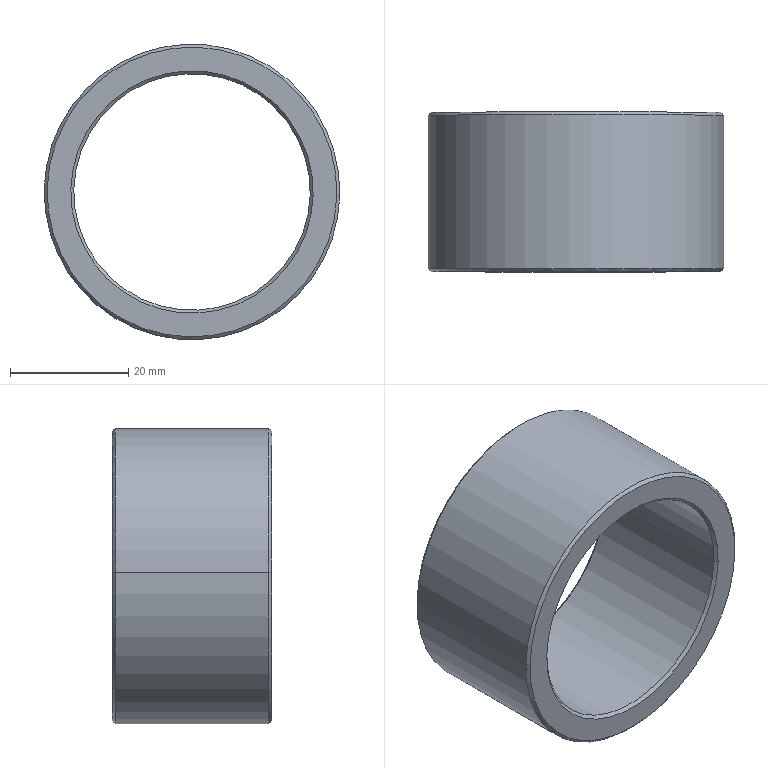Component | SolidWorks | BearingHousingAssembly-1_FixedSleeve-1 | 1 solid | 14 faces | box 50 x 27 x 50 mm | volume 19014 mm3 | cone 8 | cylinder 4 | plane 2 | commonest cylinder face diameters 40 x2 50 x2 | material Plain Carbon Steel
build123d program:
from build123d import *

# Parameters (mm, degrees)
SKETCH1_R           = 25
SKETCH1_R_2         = 20
BOSS_EXTRUDE1_DEPTH = 27
CHAMFER1_SIZE       = 0.5


with BuildPart() as part:
    # Sketch1 → Boss-Extrude1 (new body)
    with BuildSketch(Plane.XY):
        Circle(SKETCH1_R)
        Circle(SKETCH1_R_2, mode=Mode.SUBTRACT)
    extrude(amount=BOSS_EXTRUDE1_DEPTH)

    # Chamfer1
    chamfer1_edges = [part.edges().sort_by_distance(p)[0] for p in [
        (-25, 0, 0),
        (-25, 0, 27),
        (-20, 0, 0),
        (-20, 0, 27),
    ]]
    chamfer(chamfer1_edges, length=CHAMFER1_SIZE)


solid = part.part

# Placed as in the assembly
solid = solid.moved(Location((-38.666, 222.264, -6), (90, 0, 0)))
STEP:
#1=CARTESIAN_POINT('',(-0.558,7.688,-0.2605));
#2=VERTEX_POINT('',#1);
#3=CARTESIAN_POINT('',(-2.487,7.688,-0.2119));
#4=VERTEX_POINT('',#3);
#5=CARTESIAN_POINT('',(-1.522,7.688,-0.2362));
#6=DIRECTION('',(-0.,-1.,-0.));
#7=DIRECTION('',(0.9997,0.,-0.02521));
#8=AXIS2_PLACEMENT_3D('',#5,#6,#7);
#9=CIRCLE('',#8,0.9646);
#10=EDGE_CURVE('',#2,#4,#9,.T.);
#11=ORIENTED_EDGE('',*,*,#10,.F.);
#12=CARTESIAN_POINT('',(-0.5383,7.707,-0.261));
#13=VERTEX_POINT('',#12);
#14=CARTESIAN_POINT('',(-0.558,7.688,-0.2605));
#15=DIRECTION('',(0.7069,0.7071,-0.01783));
#16=VECTOR('',#15,39.37);
#17=LINE('',#14,#16);
#18=EDGE_CURVE('',#2,#13,#17,.T.);
#19=ORIENTED_EDGE('',*,*,#18,.T.);
#20=CARTESIAN_POINT('',(-2.506,7.707,-0.2114));
#21=VERTEX_POINT('',#20);
#22=CARTESIAN_POINT('',(-1.522,7.707,-0.2362));
#23=DIRECTION('',(0.,1.,0.));
#24=DIRECTION('',(0.9997,0.,-0.02521));
#25=AXIS2_PLACEMENT_3D('',#22,#23,#24);
#26=CIRCLE('',#25,0.9843);
#27=EDGE_CURVE('',#21,#13,#26,.T.);
#28=ORIENTED_EDGE('',*,*,#27,.F.);
#29=CARTESIAN_POINT('',(-2.487,7.688,-0.2119));
#30=DIRECTION('',(-0.7069,0.7071,0.01783));
#31=VECTOR('',#30,39.37);
#32=LINE('',#29,#31);
#33=EDGE_CURVE('',#4,#21,#32,.T.);
#34=ORIENTED_EDGE('',*,*,#33,.F.);
#35=EDGE_LOOP('',(#11,#19,#28,#34));
#36=FACE_OUTER_BOUND('',#35,.T.);
#37=CARTESIAN_POINT('',(-1.522,7.688,-0.2362));
#38=DIRECTION('',(0.,1.,0.));
#39=DIRECTION('',(-0.9997,0.,0.02521));
#40=AXIS2_PLACEMENT_3D('',#37,#38,#39);
#41=CONICAL_SURFACE('',#40,0.9646,0.7854);
#42=ADVANCED_FACE('',(#36),#41,.T.);
#43=CARTESIAN_POINT('',(-2.309,7.707,-0.2164));
#44=VERTEX_POINT('',#43);
#45=CARTESIAN_POINT('',(-0.7351,7.707,-0.2561));
#46=VERTEX_POINT('',#45);
#47=CARTESIAN_POINT('',(-1.522,7.707,-0.2362));
#48=DIRECTION('',(-0.,-1.,-0.));
#49=DIRECTION('',(0.9997,0.,-0.02521));
#50=AXIS2_PLACEMENT_3D('',#47,#48,#49);
#51=CIRCLE('',#50,0.7874);
#52=EDGE_CURVE('',#44,#46,#51,.T.);
#53=ORIENTED_EDGE('',*,*,#52,.F.);
#54=CARTESIAN_POINT('',(-2.329,7.688,-0.2159));
#55=VERTEX_POINT('',#54);
#56=CARTESIAN_POINT('',(-2.309,7.707,-0.2164));
#57=DIRECTION('',(-0.7069,-0.7071,0.01783));
#58=VECTOR('',#57,39.37);
#59=LINE('',#56,#58);
#60=EDGE_CURVE('',#44,#55,#59,.T.);
#61=ORIENTED_EDGE('',*,*,#60,.T.);
#62=CARTESIAN_POINT('',(-0.7154,7.688,-0.2566));
#63=VERTEX_POINT('',#62);
#64=CARTESIAN_POINT('',(-1.522,7.688,-0.2362));
#65=DIRECTION('',(0.,1.,0.));
#66=DIRECTION('',(0.9997,0.,-0.02521));
#67=AXIS2_PLACEMENT_3D('',#64,#65,#66);
#68=CIRCLE('',#67,0.8071);
#69=EDGE_CURVE('',#63,#55,#68,.T.);
#70=ORIENTED_EDGE('',*,*,#69,.F.);
#71=CARTESIAN_POINT('',(-0.7351,7.707,-0.2561));
#72=DIRECTION('',(0.7069,-0.7071,-0.01783));
#73=VECTOR('',#72,39.37);
#74=LINE('',#71,#73);
#75=EDGE_CURVE('',#46,#63,#74,.T.);
#76=ORIENTED_EDGE('',*,*,#75,.F.);
#77=EDGE_LOOP('',(#53,#61,#70,#76));
#78=FACE_OUTER_BOUND('',#77,.T.);
#79=CARTESIAN_POINT('',(-1.522,7.707,-0.2362));
#80=DIRECTION('',(-0.,-1.,-0.));
#81=DIRECTION('',(0.9997,0.,-0.02521));
#82=AXIS2_PLACEMENT_3D('',#79,#80,#81);
#83=CONICAL_SURFACE('',#82,0.7874,0.7854);
#84=ADVANCED_FACE('',(#78),#83,.F.);
#85=CARTESIAN_POINT('',(-0.7351,8.731,-0.2561));
#86=VERTEX_POINT('',#85);
#87=CARTESIAN_POINT('',(-2.309,8.731,-0.2164));
#88=VERTEX_POINT('',#87);
#89=CARTESIAN_POINT('',(-1.522,8.731,-0.2362));
#90=DIRECTION('',(0.,1.,0.));
#91=DIRECTION('',(0.9997,0.,-0.02521));
#92=AXIS2_PLACEMENT_3D('',#89,#90,#91);
#93=CIRCLE('',#92,0.7874);
#94=EDGE_CURVE('',#86,#88,#93,.T.);
#95=ORIENTED_EDGE('',*,*,#94,.F.);
#96=CARTESIAN_POINT('',(-0.7154,8.751,-0.2566));
#97=VERTEX_POINT('',#96);
#98=CARTESIAN_POINT('',(-0.7154,8.751,-0.2566));
#99=DIRECTION('',(0.7069,0.7071,-0.01783));
#100=VECTOR('',#99,39.37);
#101=LINE('',#98,#100);
#102=EDGE_CURVE('',#86,#97,#101,.T.);
#103=ORIENTED_EDGE('',*,*,#102,.T.);
#104=CARTESIAN_POINT('',(-2.329,8.751,-0.2159));
#105=VERTEX_POINT('',#104);
#106=CARTESIAN_POINT('',(-1.522,8.751,-0.2362));
#107=DIRECTION('',(-0.,-1.,-0.));
#108=DIRECTION('',(0.9997,0.,-0.02521));
#109=AXIS2_PLACEMENT_3D('',#106,#107,#108);
#110=CIRCLE('',#109,0.8071);
#111=EDGE_CURVE('',#105,#97,#110,.T.);
#112=ORIENTED_EDGE('',*,*,#111,.F.);
#113=CARTESIAN_POINT('',(-2.329,8.751,-0.2159));
#114=DIRECTION('',(-0.7069,0.7071,0.01783));
#115=VECTOR('',#114,39.37);
#116=LINE('',#113,#115);
#117=EDGE_CURVE('',#88,#105,#116,.T.);
#118=ORIENTED_EDGE('',*,*,#117,.F.);
#119=EDGE_LOOP('',(#95,#103,#112,#118));
#120=FACE_OUTER_BOUND('',#119,.T.);
#121=CARTESIAN_POINT('',(-1.522,8.751,-0.2362));
#122=DIRECTION('',(0.,1.,0.));
#123=DIRECTION('',(-0.9997,0.,0.02521));
#124=AXIS2_PLACEMENT_3D('',#121,#122,#123);
#125=CONICAL_SURFACE('',#124,0.8071,0.7854);
#126=ADVANCED_FACE('',(#120),#125,.F.);
#127=CARTESIAN_POINT('',(-2.487,8.751,-0.2119));
#128=VERTEX_POINT('',#127);
#129=CARTESIAN_POINT('',(-0.558,8.751,-0.2605));
#130=VERTEX_POINT('',#129);
#131=CARTESIAN_POINT('',(-1.522,8.751,-0.2362));
#132=DIRECTION('',(0.,1.,0.));
#133=DIRECTION('',(0.9997,0.,-0.02521));
#134=AXIS2_PLACEMENT_3D('',#131,#132,#133);
#135=CIRCLE('',#134,0.9646);
#136=EDGE_CURVE('',#128,#130,#135,.T.);
#137=ORIENTED_EDGE('',*,*,#136,.F.);
#138=CARTESIAN_POINT('',(-2.506,8.731,-0.2114));
#139=VERTEX_POINT('',#138);
#140=CARTESIAN_POINT('',(-2.506,8.731,-0.2114));
#141=DIRECTION('',(-0.7069,-0.7071,0.01783));
#142=VECTOR('',#141,39.37);
#143=LINE('',#140,#142);
#144=EDGE_CURVE('',#128,#139,#143,.T.);
#145=ORIENTED_EDGE('',*,*,#144,.T.);
#146=CARTESIAN_POINT('',(-0.5383,8.731,-0.261));
#147=VERTEX_POINT('',#146);
#148=CARTESIAN_POINT('',(-1.522,8.731,-0.2362));
#149=DIRECTION('',(-0.,-1.,-0.));
#150=DIRECTION('',(0.9997,0.,-0.02521));
#151=AXIS2_PLACEMENT_3D('',#148,#149,#150);
#152=CIRCLE('',#151,0.9843);
#153=EDGE_CURVE('',#147,#139,#152,.T.);
#154=ORIENTED_EDGE('',*,*,#153,.F.);
#155=CARTESIAN_POINT('',(-0.5383,8.731,-0.261));
#156=DIRECTION('',(0.7069,-0.7071,-0.01783));
#157=VECTOR('',#156,39.37);
#158=LINE('',#155,#157);
#159=EDGE_CURVE('',#130,#147,#158,.T.);
#160=ORIENTED_EDGE('',*,*,#159,.F.);
#161=EDGE_LOOP('',(#137,#145,#154,#160));
#162=FACE_OUTER_BOUND('',#161,.T.);
#163=CARTESIAN_POINT('',(-1.522,8.731,-0.2362));
#164=DIRECTION('',(-0.,-1.,-0.));
#165=DIRECTION('',(0.9997,0.,-0.02521));
#166=AXIS2_PLACEMENT_3D('',#163,#164,#165);
#167=CONICAL_SURFACE('',#166,0.9843,0.7854);
#168=ADVANCED_FACE('',(#162),#167,.T.);
#169=ORIENTED_EDGE('',*,*,#52,.T.);
#170=CARTESIAN_POINT('',(-0.7351,7.688,-0.2561));
#171=DIRECTION('',(0.,1.,0.));
#172=VECTOR('',#171,39.37);
#173=LINE('',#170,#172);
#174=EDGE_CURVE('',#46,#86,#173,.T.);
#175=ORIENTED_EDGE('',*,*,#174,.T.);
#176=ORIENTED_EDGE('',*,*,#94,.T.);
#177=CARTESIAN_POINT('',(-2.309,7.688,-0.2164));
#178=DIRECTION('',(0.,1.,0.));
#179=VECTOR('',#178,39.37);
#180=LINE('',#177,#179);
#181=EDGE_CURVE('',#44,#88,#180,.T.);
#182=ORIENTED_EDGE('',*,*,#181,.F.);
#183=EDGE_LOOP('',(#169,#175,#176,#182));
#184=FACE_OUTER_BOUND('',#183,.T.);
#185=CARTESIAN_POINT('',(-1.522,7.688,-0.2362));
#186=DIRECTION('',(0.,1.,0.));
#187=DIRECTION('',(-0.9997,0.,0.02521));
#188=AXIS2_PLACEMENT_3D('',#185,#186,#187);
#189=CYLINDRICAL_SURFACE('',#188,0.7874);
#190=ADVANCED_FACE('',(#184),#189,.F.);
#191=ORIENTED_EDGE('',*,*,#27,.T.);
#192=CARTESIAN_POINT('',(-0.5383,7.688,-0.261));
#193=DIRECTION('',(0.,1.,0.));
#194=VECTOR('',#193,39.37);
#195=LINE('',#192,#194);
#196=EDGE_CURVE('',#13,#147,#195,.T.);
#197=ORIENTED_EDGE('',*,*,#196,.T.);
#198=ORIENTED_EDGE('',*,*,#153,.T.);
#199=CARTESIAN_POINT('',(-2.506,7.688,-0.2114));
#200=DIRECTION('',(0.,1.,0.));
#201=VECTOR('',#200,39.37);
#202=LINE('',#199,#201);
#203=EDGE_CURVE('',#21,#139,#202,.T.);
#204=ORIENTED_EDGE('',*,*,#203,.F.);
#205=EDGE_LOOP('',(#191,#197,#198,#204));
#206=FACE_OUTER_BOUND('',#205,.T.);
#207=CARTESIAN_POINT('',(-1.522,7.688,-0.2362));
#208=DIRECTION('',(0.,1.,0.));
#209=DIRECTION('',(-0.9997,0.,0.02521));
#210=AXIS2_PLACEMENT_3D('',#207,#208,#209);
#211=CYLINDRICAL_SURFACE('',#210,0.9843);
#212=ADVANCED_FACE('',(#206),#211,.T.);
#213=ORIENTED_EDGE('',*,*,#69,.T.);
#214=CARTESIAN_POINT('',(-1.522,7.688,-0.2362));
#215=DIRECTION('',(0.,1.,0.));
#216=DIRECTION('',(0.9997,0.,-0.02521));
#217=AXIS2_PLACEMENT_3D('',#214,#215,#216);
#218=CIRCLE('',#217,0.8071);
#219=EDGE_CURVE('',#55,#63,#218,.T.);
#220=ORIENTED_EDGE('',*,*,#219,.T.);
#221=EDGE_LOOP('',(#213,#220));
#222=FACE_BOUND('',#221,.T.);
#223=CARTESIAN_POINT('',(-1.522,7.688,-0.2362));
#224=DIRECTION('',(-0.,-1.,-0.));
#225=DIRECTION('',(0.9997,0.,-0.02521));
#226=AXIS2_PLACEMENT_3D('',#223,#224,#225);
#227=CIRCLE('',#226,0.9646);
#228=EDGE_CURVE('',#4,#2,#227,.T.);
#229=ORIENTED_EDGE('',*,*,#228,.T.);
#230=ORIENTED_EDGE('',*,*,#10,.T.);
#231=EDGE_LOOP('',(#229,#230));
#232=FACE_OUTER_BOUND('',#231,.T.);
#233=CARTESIAN_POINT('',(-1.522,7.688,-0.2362));
#234=DIRECTION('',(-0.,-1.,-0.));
#235=DIRECTION('',(0.9997,-0.,-0.02521));
#236=AXIS2_PLACEMENT_3D('',#233,#234,#235);
#237=PLANE('',#236);
#238=ADVANCED_FACE('',(#222,#232),#237,.T.);
#239=CARTESIAN_POINT('',(-1.522,8.751,-0.2362));
#240=DIRECTION('',(0.,1.,0.));
#241=DIRECTION('',(0.9997,0.,-0.02521));
#242=AXIS2_PLACEMENT_3D('',#239,#240,#241);
#243=CIRCLE('',#242,0.9646);
#244=EDGE_CURVE('',#130,#128,#243,.T.);
#245=ORIENTED_EDGE('',*,*,#244,.T.);
#246=ORIENTED_EDGE('',*,*,#136,.T.);
#247=EDGE_LOOP('',(#245,#246));
#248=FACE_OUTER_BOUND('',#247,.T.);
#249=ORIENTED_EDGE('',*,*,#111,.T.);
#250=CARTESIAN_POINT('',(-1.522,8.751,-0.2362));
#251=DIRECTION('',(-0.,-1.,-0.));
#252=DIRECTION('',(0.9997,0.,-0.02521));
#253=AXIS2_PLACEMENT_3D('',#250,#251,#252);
#254=CIRCLE('',#253,0.8071);
#255=EDGE_CURVE('',#97,#105,#254,.T.);
#256=ORIENTED_EDGE('',*,*,#255,.T.);
#257=EDGE_LOOP('',(#249,#256));
#258=FACE_BOUND('',#257,.T.);
#259=CARTESIAN_POINT('',(-1.522,8.751,-0.2362));
#260=DIRECTION('',(-0.,-1.,-0.));
#261=DIRECTION('',(0.9997,-0.,-0.02521));
#262=AXIS2_PLACEMENT_3D('',#259,#260,#261);
#263=PLANE('',#262);
#264=ADVANCED_FACE('',(#248,#258),#263,.F.);
#265=ORIENTED_EDGE('',*,*,#196,.F.);
#266=CARTESIAN_POINT('',(-1.522,7.707,-0.2362));
#267=DIRECTION('',(0.,1.,0.));
#268=DIRECTION('',(0.9997,0.,-0.02521));
#269=AXIS2_PLACEMENT_3D('',#266,#267,#268);
#270=CIRCLE('',#269,0.9843);
#271=EDGE_CURVE('',#13,#21,#270,.T.);
#272=ORIENTED_EDGE('',*,*,#271,.T.);
#273=ORIENTED_EDGE('',*,*,#203,.T.);
#274=CARTESIAN_POINT('',(-1.522,8.731,-0.2362));
#275=DIRECTION('',(-0.,-1.,-0.));
#276=DIRECTION('',(0.9997,0.,-0.02521));
#277=AXIS2_PLACEMENT_3D('',#274,#275,#276);
#278=CIRCLE('',#277,0.9843);
#279=EDGE_CURVE('',#139,#147,#278,.T.);
#280=ORIENTED_EDGE('',*,*,#279,.T.);
#281=EDGE_LOOP('',(#265,#272,#273,#280));
#282=FACE_OUTER_BOUND('',#281,.T.);
#283=CARTESIAN_POINT('',(-1.522,7.688,-0.2362));
#284=DIRECTION('',(0.,1.,0.));
#285=DIRECTION('',(-0.9997,0.,0.02521));
#286=AXIS2_PLACEMENT_3D('',#283,#284,#285);
#287=CYLINDRICAL_SURFACE('',#286,0.9843);
#288=ADVANCED_FACE('',(#282),#287,.T.);
#289=ORIENTED_EDGE('',*,*,#174,.F.);
#290=CARTESIAN_POINT('',(-1.522,7.707,-0.2362));
#291=DIRECTION('',(-0.,-1.,-0.));
#292=DIRECTION('',(0.9997,0.,-0.02521));
#293=AXIS2_PLACEMENT_3D('',#290,#291,#292);
#294=CIRCLE('',#293,0.7874);
#295=EDGE_CURVE('',#46,#44,#294,.T.);
#296=ORIENTED_EDGE('',*,*,#295,.T.);
#297=ORIENTED_EDGE('',*,*,#181,.T.);
#298=CARTESIAN_POINT('',(-1.522,8.731,-0.2362));
#299=DIRECTION('',(0.,1.,0.));
#300=DIRECTION('',(0.9997,0.,-0.02521));
#301=AXIS2_PLACEMENT_3D('',#298,#299,#300);
#302=CIRCLE('',#301,0.7874);
#303=EDGE_CURVE('',#88,#86,#302,.T.);
#304=ORIENTED_EDGE('',*,*,#303,.T.);
#305=EDGE_LOOP('',(#289,#296,#297,#304));
#306=FACE_OUTER_BOUND('',#305,.T.);
#307=CARTESIAN_POINT('',(-1.522,7.688,-0.2362));
#308=DIRECTION('',(0.,1.,0.));
#309=DIRECTION('',(-0.9997,0.,0.02521));
#310=AXIS2_PLACEMENT_3D('',#307,#308,#309);
#311=CYLINDRICAL_SURFACE('',#310,0.7874);
#312=ADVANCED_FACE('',(#306),#311,.F.);
#313=ORIENTED_EDGE('',*,*,#144,.F.);
#314=ORIENTED_EDGE('',*,*,#244,.F.);
#315=ORIENTED_EDGE('',*,*,#159,.T.);
#316=ORIENTED_EDGE('',*,*,#279,.F.);
#317=EDGE_LOOP('',(#313,#314,#315,#316));
#318=FACE_OUTER_BOUND('',#317,.T.);
#319=CARTESIAN_POINT('',(-1.522,8.731,-0.2362));
#320=DIRECTION('',(-0.,-1.,-0.));
#321=DIRECTION('',(0.9997,0.,-0.02521));
#322=AXIS2_PLACEMENT_3D('',#319,#320,#321);
#323=CONICAL_SURFACE('',#322,0.9843,0.7854);
#324=ADVANCED_FACE('',(#318),#323,.T.);
#325=ORIENTED_EDGE('',*,*,#102,.F.);
#326=ORIENTED_EDGE('',*,*,#303,.F.);
#327=ORIENTED_EDGE('',*,*,#117,.T.);
#328=ORIENTED_EDGE('',*,*,#255,.F.);
#329=EDGE_LOOP('',(#325,#326,#327,#328));
#330=FACE_OUTER_BOUND('',#329,.T.);
#331=CARTESIAN_POINT('',(-1.522,8.751,-0.2362));
#332=DIRECTION('',(0.,1.,0.));
#333=DIRECTION('',(-0.9997,0.,0.02521));
#334=AXIS2_PLACEMENT_3D('',#331,#332,#333);
#335=CONICAL_SURFACE('',#334,0.8071,0.7854);
#336=ADVANCED_FACE('',(#330),#335,.F.);
#337=ORIENTED_EDGE('',*,*,#60,.F.);
#338=ORIENTED_EDGE('',*,*,#295,.F.);
#339=ORIENTED_EDGE('',*,*,#75,.T.);
#340=ORIENTED_EDGE('',*,*,#219,.F.);
#341=EDGE_LOOP('',(#337,#338,#339,#340));
#342=FACE_OUTER_BOUND('',#341,.T.);
#343=CARTESIAN_POINT('',(-1.522,7.707,-0.2362));
#344=DIRECTION('',(-0.,-1.,-0.));
#345=DIRECTION('',(0.9997,0.,-0.02521));
#346=AXIS2_PLACEMENT_3D('',#343,#344,#345);
#347=CONICAL_SURFACE('',#346,0.7874,0.7854);
#348=ADVANCED_FACE('',(#342),#347,.F.);
#349=ORIENTED_EDGE('',*,*,#18,.F.);
#350=ORIENTED_EDGE('',*,*,#228,.F.);
#351=ORIENTED_EDGE('',*,*,#33,.T.);
#352=ORIENTED_EDGE('',*,*,#271,.F.);
#353=EDGE_LOOP('',(#349,#350,#351,#352));
#354=FACE_OUTER_BOUND('',#353,.T.);
#355=CARTESIAN_POINT('',(-1.522,7.688,-0.2362));
#356=DIRECTION('',(0.,1.,0.));
#357=DIRECTION('',(-0.9997,0.,0.02521));
#358=AXIS2_PLACEMENT_3D('',#355,#356,#357);
#359=CONICAL_SURFACE('',#358,0.9646,0.7854);
#360=ADVANCED_FACE('',(#354),#359,.T.);
#361=CLOSED_SHELL('',(#42,#84,#126,#168,#190,#212,#238,#264,#288,#312,#324,#336,#348,#360));
#362=MANIFOLD_SOLID_BREP('',#361);
#363=CARTESIAN_POINT('',(0.,0.,0.));
#364=DIRECTION('',(0.,0.,1.));
#365=DIRECTION('',(1.,0.,0.));
#366=AXIS2_PLACEMENT_3D('',#363,#364,#365);
#367=(LENGTH_UNIT()NAMED_UNIT(*)SI_UNIT($,.METRE.));
#368=LENGTH_MEASURE_WITH_UNIT(LENGTH_MEASURE(0.0254),#367);
#369=DIMENSIONAL_EXPONENTS(1.,0.,0.,0.,0.,0.,0.);
#370=(CONVERSION_BASED_UNIT('',#368)LENGTH_UNIT()NAMED_UNIT(#369));
#371=UNCERTAINTY_MEASURE_WITH_UNIT(LENGTH_MEASURE(0.00001),#370,'','');
#372=(NAMED_UNIT(*)PLANE_ANGLE_UNIT()SI_UNIT($,.RADIAN.));
#373=(NAMED_UNIT(*)SI_UNIT($,.STERADIAN.)SOLID_ANGLE_UNIT());
#374=(GEOMETRIC_REPRESENTATION_CONTEXT(3)GLOBAL_UNCERTAINTY_ASSIGNED_CONTEXT((#371))GLOBAL_UNIT_ASSIGNED_CONTEXT((#370,#372,#373))REPRESENTATION_CONTEXT('',''));
#375=ADVANCED_BREP_SHAPE_REPRESENTATION('',(#362,#366),#374);
#376=COLOUR_RGB('',0.7922,0.8196,0.9333);
#377=FILL_AREA_STYLE_COLOUR('',#376);
#378=FILL_AREA_STYLE('',(#377));
#379=SURFACE_STYLE_FILL_AREA(#378);
#380=SURFACE_SIDE_STYLE('',(#379));
#381=SURFACE_STYLE_USAGE(.BOTH.,#380);
#382=PRESENTATION_STYLE_ASSIGNMENT((#381));
#383=STYLED_ITEM('',(#382),#362);
#384=(LENGTH_UNIT()NAMED_UNIT(*)SI_UNIT($,.METRE.));
#385=LENGTH_MEASURE_WITH_UNIT(LENGTH_MEASURE(0.0254),#384);
#386=DIMENSIONAL_EXPONENTS(1.,0.,0.,0.,0.,0.,0.);
#387=(CONVERSION_BASED_UNIT('',#385)LENGTH_UNIT()NAMED_UNIT(#386));
#388=UNCERTAINTY_MEASURE_WITH_UNIT(LENGTH_MEASURE(0.00001),#387,'','');
#389=(NAMED_UNIT(*)PLANE_ANGLE_UNIT()SI_UNIT($,.RADIAN.));
#390=(NAMED_UNIT(*)SI_UNIT($,.STERADIAN.)SOLID_ANGLE_UNIT());
#391=(GEOMETRIC_REPRESENTATION_CONTEXT(3)GLOBAL_UNCERTAINTY_ASSIGNED_CONTEXT((#388))GLOBAL_UNIT_ASSIGNED_CONTEXT((#387,#389,#390))REPRESENTATION_CONTEXT('',''));
#392=MECHANICAL_DESIGN_GEOMETRIC_PRESENTATION_REPRESENTATION('',(#383),#391);
#393=PRESENTATION_LAYER_ASSIGNMENT('','',(#383));